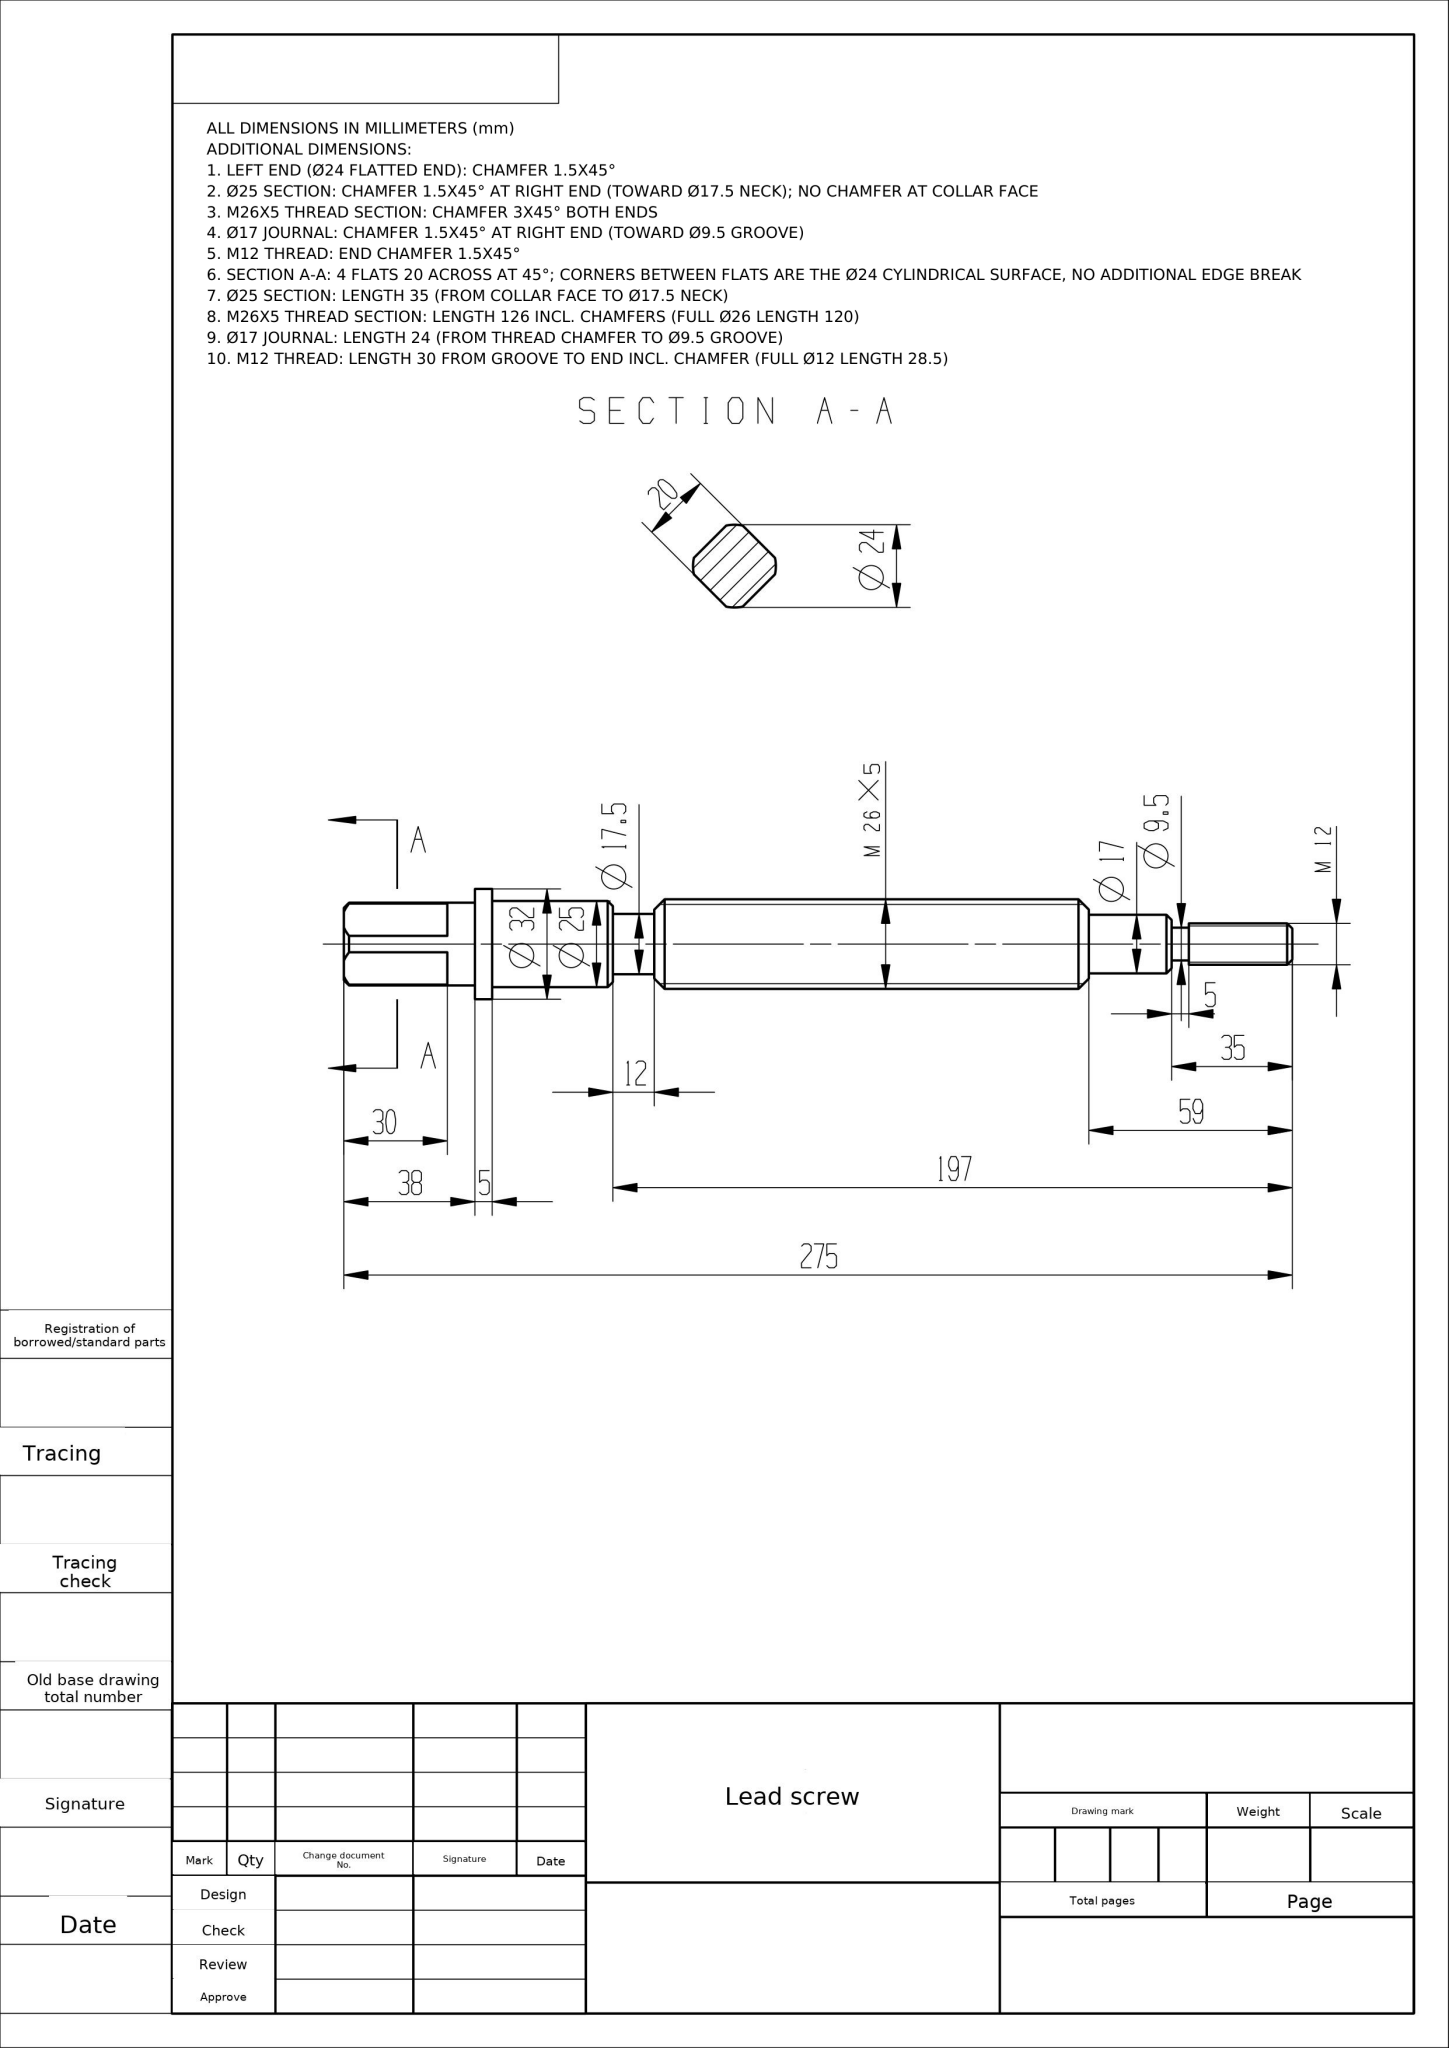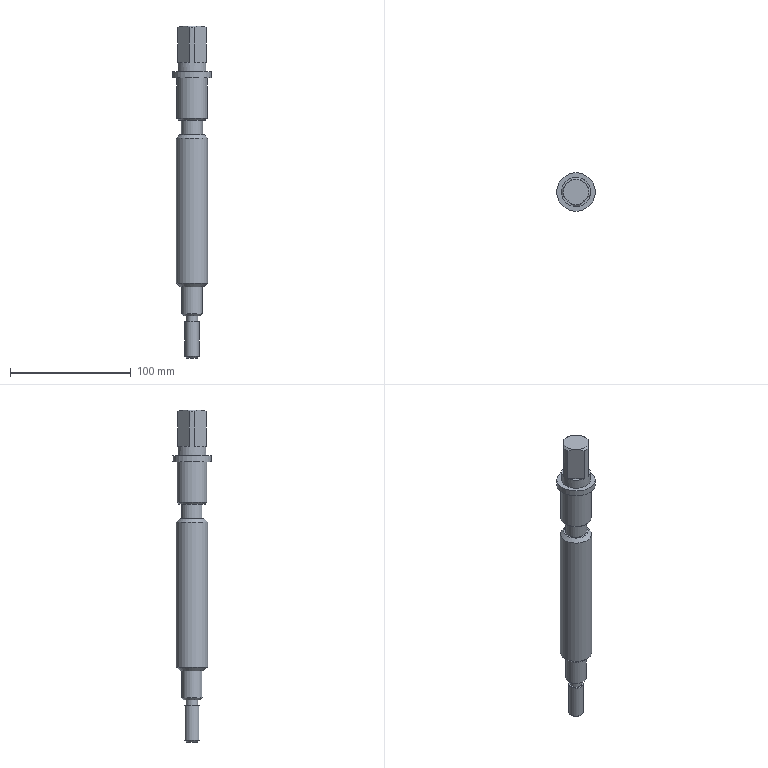Part | NX | mm | 1 solid | 34 faces | box 32 x 32 x 275 mm | volume 114323 mm3 | plane 17 | cone 9 | cylinder 8 | commonest cylinder face diameters 17.5 x1 25 x1 24 x1 32 x1 26 x1 12 x1 9.5 x1 17 x1
STEP:
#1=CARTESIAN_POINT('',(0.,0.,0.));
#2=DIRECTION('',(0.,0.,1.));
#3=DIRECTION('',(1.,0.,0.));
#4=AXIS2_PLACEMENT_3D('',#1,#2,#3);
#5=(LENGTH_UNIT()NAMED_UNIT(*)SI_UNIT(.MILLI.,.METRE.));
#6=UNCERTAINTY_MEASURE_WITH_UNIT(LENGTH_MEASURE(0.0508),#5,'','');
#7=(NAMED_UNIT(*)PLANE_ANGLE_UNIT()SI_UNIT($,.RADIAN.));
#8=PLANE_ANGLE_MEASURE_WITH_UNIT(PLANE_ANGLE_MEASURE(0.01745),#7);
#9=DIMENSIONAL_EXPONENTS(0.,0.,0.,0.,0.,0.,0.);
#10=(CONVERSION_BASED_UNIT('',#8)NAMED_UNIT(#9)PLANE_ANGLE_UNIT());
#11=(NAMED_UNIT(*)SI_UNIT($,.STERADIAN.)SOLID_ANGLE_UNIT());
#12=(GEOMETRIC_REPRESENTATION_CONTEXT(3)GLOBAL_UNCERTAINTY_ASSIGNED_CONTEXT((#6))GLOBAL_UNIT_ASSIGNED_CONTEXT((#5,#10,#11))REPRESENTATION_CONTEXT('',''));
#13=SHAPE_REPRESENTATION('',(#4),#12);
#14=CARTESIAN_POINT('',(11.,0.,155.));
#15=VERTEX_POINT('',#14);
#16=CARTESIAN_POINT('',(0.,0.,155.));
#17=DIRECTION('',(0.,0.,-1.));
#18=DIRECTION('',(1.,0.,0.));
#19=AXIS2_PLACEMENT_3D('',#16,#17,#18);
#20=CIRCLE('',#19,11.);
#21=EDGE_CURVE('',#15,#15,#20,.T.);
#22=ORIENTED_EDGE('',*,*,#21,.T.);
#23=EDGE_LOOP('',(#22));
#24=FACE_BOUND('',#23,.T.);
#25=CARTESIAN_POINT('',(8.75,0.,155.));
#26=VERTEX_POINT('',#25);
#27=CARTESIAN_POINT('',(0.,0.,155.));
#28=DIRECTION('',(0.,0.,-1.));
#29=DIRECTION('',(1.,0.,0.));
#30=AXIS2_PLACEMENT_3D('',#27,#28,#29);
#31=CIRCLE('',#30,8.75);
#32=EDGE_CURVE('',#26,#26,#31,.T.);
#33=ORIENTED_EDGE('',*,*,#32,.F.);
#34=EDGE_LOOP('',(#33));
#35=FACE_BOUND('',#34,.T.);
#36=CARTESIAN_POINT('',(0.,0.,155.));
#37=DIRECTION('',(0.,0.,1.));
#38=DIRECTION('',(1.,0.,0.));
#39=AXIS2_PLACEMENT_3D('',#36,#37,#38);
#40=PLANE('',#39);
#41=ADVANCED_FACE('',(#24,#35),#40,.F.);
#42=CARTESIAN_POINT('',(10.,0.,143.));
#43=VERTEX_POINT('',#42);
#44=CARTESIAN_POINT('',(0.,0.,143.));
#45=DIRECTION('',(0.,0.,1.));
#46=DIRECTION('',(1.,0.,0.));
#47=AXIS2_PLACEMENT_3D('',#44,#45,#46);
#48=CIRCLE('',#47,10.);
#49=EDGE_CURVE('',#43,#43,#48,.T.);
#50=ORIENTED_EDGE('',*,*,#49,.T.);
#51=EDGE_LOOP('',(#50));
#52=FACE_BOUND('',#51,.T.);
#53=CARTESIAN_POINT('',(8.75,0.,143.));
#54=VERTEX_POINT('',#53);
#55=CARTESIAN_POINT('',(0.,0.,143.));
#56=DIRECTION('',(0.,0.,-1.));
#57=DIRECTION('',(1.,0.,0.));
#58=AXIS2_PLACEMENT_3D('',#55,#56,#57);
#59=CIRCLE('',#58,8.75);
#60=EDGE_CURVE('',#54,#54,#59,.T.);
#61=ORIENTED_EDGE('',*,*,#60,.T.);
#62=EDGE_LOOP('',(#61));
#63=FACE_BOUND('',#62,.T.);
#64=CARTESIAN_POINT('',(0.,0.,143.));
#65=DIRECTION('',(0.,0.,1.));
#66=DIRECTION('',(1.,0.,0.));
#67=AXIS2_PLACEMENT_3D('',#64,#65,#66);
#68=PLANE('',#67);
#69=ADVANCED_FACE('',(#52,#63),#68,.T.);
#70=ORIENTED_EDGE('',*,*,#32,.T.);
#71=EDGE_LOOP('',(#70));
#72=FACE_BOUND('',#71,.T.);
#73=ORIENTED_EDGE('',*,*,#60,.F.);
#74=EDGE_LOOP('',(#73));
#75=FACE_BOUND('',#74,.T.);
#76=CARTESIAN_POINT('',(0.,0.,155.));
#77=DIRECTION('',(0.,0.,-1.));
#78=DIRECTION('',(-1.,0.,0.));
#79=AXIS2_PLACEMENT_3D('',#76,#77,#78);
#80=CYLINDRICAL_SURFACE('',#79,8.75);
#81=ADVANCED_FACE('',(#72,#75),#80,.T.);
#82=CARTESIAN_POINT('',(12.5,0.,156.5));
#83=VERTEX_POINT('',#82);
#84=CARTESIAN_POINT('',(0.,0.,156.5));
#85=DIRECTION('',(0.,0.,1.));
#86=DIRECTION('',(1.,0.,0.));
#87=AXIS2_PLACEMENT_3D('',#84,#85,#86);
#88=CIRCLE('',#87,12.5);
#89=EDGE_CURVE('',#83,#83,#88,.T.);
#90=ORIENTED_EDGE('',*,*,#89,.T.);
#91=EDGE_LOOP('',(#90));
#92=FACE_BOUND('',#91,.T.);
#93=CARTESIAN_POINT('',(12.5,0.,190.));
#94=VERTEX_POINT('',#93);
#95=CARTESIAN_POINT('',(0.,0.,190.));
#96=DIRECTION('',(0.,0.,-1.));
#97=DIRECTION('',(1.,0.,0.));
#98=AXIS2_PLACEMENT_3D('',#95,#96,#97);
#99=CIRCLE('',#98,12.5);
#100=EDGE_CURVE('',#94,#94,#99,.T.);
#101=ORIENTED_EDGE('',*,*,#100,.T.);
#102=EDGE_LOOP('',(#101));
#103=FACE_BOUND('',#102,.T.);
#104=CARTESIAN_POINT('',(0.,0.,155.));
#105=DIRECTION('',(0.,0.,1.));
#106=DIRECTION('',(1.,0.,0.));
#107=AXIS2_PLACEMENT_3D('',#104,#105,#106);
#108=CYLINDRICAL_SURFACE('',#107,12.5);
#109=ADVANCED_FACE('',(#92,#103),#108,.T.);
#110=CARTESIAN_POINT('',(-9.335,4.807,233.));
#111=VERTEX_POINT('',#110);
#112=CARTESIAN_POINT('',(-4.807,9.335,233.));
#113=VERTEX_POINT('',#112);
#114=CARTESIAN_POINT('',(-11.761,2.381,233.));
#115=DIRECTION('',(0.7071,0.7071,0.));
#116=VECTOR('',#115,1.);
#117=LINE('',#114,#116);
#118=EDGE_CURVE('',#111,#113,#117,.T.);
#119=ORIENTED_EDGE('',*,*,#118,.F.);
#120=CARTESIAN_POINT('',(-9.335,-4.807,233.));
#121=VERTEX_POINT('',#120);
#122=CARTESIAN_POINT('',(0.,0.,233.));
#123=DIRECTION('',(0.,0.,1.));
#124=DIRECTION('',(1.,0.,0.));
#125=AXIS2_PLACEMENT_3D('',#122,#123,#124);
#126=CIRCLE('',#125,10.5);
#127=EDGE_CURVE('',#111,#121,#126,.T.);
#128=ORIENTED_EDGE('',*,*,#127,.T.);
#129=CARTESIAN_POINT('',(-4.807,-9.335,233.));
#130=VERTEX_POINT('',#129);
#131=CARTESIAN_POINT('',(-2.381,-11.761,233.));
#132=DIRECTION('',(-0.7071,0.7071,0.));
#133=VECTOR('',#132,1.);
#134=LINE('',#131,#133);
#135=EDGE_CURVE('',#130,#121,#134,.T.);
#136=ORIENTED_EDGE('',*,*,#135,.F.);
#137=CARTESIAN_POINT('',(4.807,-9.335,233.));
#138=VERTEX_POINT('',#137);
#139=CARTESIAN_POINT('',(0.,0.,233.));
#140=DIRECTION('',(0.,0.,1.));
#141=DIRECTION('',(1.,0.,0.));
#142=AXIS2_PLACEMENT_3D('',#139,#140,#141);
#143=CIRCLE('',#142,10.5);
#144=EDGE_CURVE('',#130,#138,#143,.T.);
#145=ORIENTED_EDGE('',*,*,#144,.T.);
#146=CARTESIAN_POINT('',(9.335,-4.807,233.));
#147=VERTEX_POINT('',#146);
#148=CARTESIAN_POINT('',(11.761,-2.381,233.));
#149=DIRECTION('',(-0.7071,-0.7071,0.));
#150=VECTOR('',#149,1.);
#151=LINE('',#148,#150);
#152=EDGE_CURVE('',#147,#138,#151,.T.);
#153=ORIENTED_EDGE('',*,*,#152,.F.);
#154=CARTESIAN_POINT('',(9.335,4.807,233.));
#155=VERTEX_POINT('',#154);
#156=CARTESIAN_POINT('',(0.,0.,233.));
#157=DIRECTION('',(0.,0.,1.));
#158=DIRECTION('',(1.,0.,0.));
#159=AXIS2_PLACEMENT_3D('',#156,#157,#158);
#160=CIRCLE('',#159,10.5);
#161=EDGE_CURVE('',#147,#155,#160,.T.);
#162=ORIENTED_EDGE('',*,*,#161,.T.);
#163=CARTESIAN_POINT('',(4.807,9.335,233.));
#164=VERTEX_POINT('',#163);
#165=CARTESIAN_POINT('',(2.381,11.761,233.));
#166=DIRECTION('',(0.7071,-0.7071,0.));
#167=VECTOR('',#166,1.);
#168=LINE('',#165,#167);
#169=EDGE_CURVE('',#164,#155,#168,.T.);
#170=ORIENTED_EDGE('',*,*,#169,.F.);
#171=CARTESIAN_POINT('',(0.,0.,233.));
#172=DIRECTION('',(0.,0.,1.));
#173=DIRECTION('',(1.,0.,0.));
#174=AXIS2_PLACEMENT_3D('',#171,#172,#173);
#175=CIRCLE('',#174,10.5);
#176=EDGE_CURVE('',#164,#113,#175,.T.);
#177=ORIENTED_EDGE('',*,*,#176,.T.);
#178=EDGE_LOOP('',(#119,#128,#136,#145,#153,#162,#170,#177));
#179=FACE_OUTER_BOUND('',#178,.T.);
#180=CARTESIAN_POINT('',(0.,0.,233.));
#181=DIRECTION('',(0.,0.,1.));
#182=DIRECTION('',(1.,0.,0.));
#183=AXIS2_PLACEMENT_3D('',#180,#181,#182);
#184=PLANE('',#183);
#185=ADVANCED_FACE('',(#179),#184,.T.);
#186=CARTESIAN_POINT('',(-11.761,2.381,231.5));
#187=VERTEX_POINT('',#186);
#188=CARTESIAN_POINT('',(-11.761,2.381,231.5));
#189=CARTESIAN_POINT('',(-10.993,3.15,232.101));
#190=CARTESIAN_POINT('',(-10.184,3.958,232.634));
#191=CARTESIAN_POINT('',(-9.335,4.807,233.));
#192=B_SPLINE_CURVE_WITH_KNOTS('',3,(#188,#189,#190,#191),.UNSPECIFIED.,.F.,.F.,(4,4),(0.,1.),.UNSPECIFIED.);
#193=EDGE_CURVE('',#187,#111,#192,.T.);
#194=ORIENTED_EDGE('',*,*,#193,.F.);
#195=CARTESIAN_POINT('',(-11.761,-2.381,231.5));
#196=VERTEX_POINT('',#195);
#197=CARTESIAN_POINT('',(0.,0.,231.5));
#198=DIRECTION('',(0.,0.,-1.));
#199=DIRECTION('',(1.,0.,0.));
#200=AXIS2_PLACEMENT_3D('',#197,#198,#199);
#201=CIRCLE('',#200,12.);
#202=EDGE_CURVE('',#196,#187,#201,.T.);
#203=ORIENTED_EDGE('',*,*,#202,.F.);
#204=CARTESIAN_POINT('',(-9.335,-4.807,233.));
#205=CARTESIAN_POINT('',(-10.178,-3.964,232.636));
#206=CARTESIAN_POINT('',(-10.993,-3.149,232.101));
#207=CARTESIAN_POINT('',(-11.761,-2.381,231.5));
#208=B_SPLINE_CURVE_WITH_KNOTS('',3,(#204,#205,#206,#207),.UNSPECIFIED.,.F.,.F.,(4,4),(0.,1.),.UNSPECIFIED.);
#209=EDGE_CURVE('',#121,#196,#208,.T.);
#210=ORIENTED_EDGE('',*,*,#209,.F.);
#211=ORIENTED_EDGE('',*,*,#127,.F.);
#212=EDGE_LOOP('',(#194,#203,#210,#211));
#213=FACE_OUTER_BOUND('',#212,.T.);
#214=CARTESIAN_POINT('',(0.,0.,233.));
#215=DIRECTION('',(0.,0.,-1.));
#216=DIRECTION('',(-1.,0.,-0.));
#217=AXIS2_PLACEMENT_3D('',#214,#215,#216);
#218=CONICAL_SURFACE('',#217,10.5,45.);
#219=ADVANCED_FACE('',(#213),#218,.T.);
#220=CARTESIAN_POINT('',(-11.761,-2.381,203.));
#221=VERTEX_POINT('',#220);
#222=CARTESIAN_POINT('',(-2.381,-11.761,203.));
#223=VERTEX_POINT('',#222);
#224=CARTESIAN_POINT('',(-2.381,-11.761,203.));
#225=DIRECTION('',(0.7071,-0.7071,0.));
#226=VECTOR('',#225,1.);
#227=LINE('',#224,#226);
#228=EDGE_CURVE('',#221,#223,#227,.T.);
#229=ORIENTED_EDGE('',*,*,#228,.F.);
#230=CARTESIAN_POINT('',(0.,0.,203.));
#231=DIRECTION('',(0.,0.,1.));
#232=DIRECTION('',(-1.,-0.,0.));
#233=AXIS2_PLACEMENT_3D('',#230,#231,#232);
#234=CIRCLE('',#233,12.);
#235=EDGE_CURVE('',#221,#223,#234,.T.);
#236=ORIENTED_EDGE('',*,*,#235,.T.);
#237=EDGE_LOOP('',(#229,#236));
#238=FACE_OUTER_BOUND('',#237,.T.);
#239=CARTESIAN_POINT('',(0.,0.,203.));
#240=DIRECTION('',(0.,0.,1.));
#241=DIRECTION('',(-1.,-0.,0.));
#242=AXIS2_PLACEMENT_3D('',#239,#240,#241);
#243=PLANE('',#242);
#244=ADVANCED_FACE('',(#238),#243,.T.);
#245=CARTESIAN_POINT('',(-2.381,-11.761,231.5));
#246=VERTEX_POINT('',#245);
#247=CARTESIAN_POINT('',(-2.381,-11.761,231.5));
#248=CARTESIAN_POINT('',(-3.15,-10.993,232.101));
#249=CARTESIAN_POINT('',(-3.958,-10.184,232.634));
#250=CARTESIAN_POINT('',(-4.807,-9.335,233.));
#251=B_SPLINE_CURVE_WITH_KNOTS('',3,(#247,#248,#249,#250),.UNSPECIFIED.,.F.,.F.,(4,4),(0.,1.),.UNSPECIFIED.);
#252=EDGE_CURVE('',#246,#130,#251,.T.);
#253=ORIENTED_EDGE('',*,*,#252,.T.);
#254=ORIENTED_EDGE('',*,*,#135,.T.);
#255=ORIENTED_EDGE('',*,*,#209,.T.);
#256=CARTESIAN_POINT('',(-11.761,-2.381,203.));
#257=DIRECTION('',(0.,0.,1.));
#258=VECTOR('',#257,1.);
#259=LINE('',#256,#258);
#260=EDGE_CURVE('',#221,#196,#259,.T.);
#261=ORIENTED_EDGE('',*,*,#260,.F.);
#262=ORIENTED_EDGE('',*,*,#228,.T.);
#263=CARTESIAN_POINT('',(-2.381,-11.761,203.));
#264=DIRECTION('',(0.,0.,-1.));
#265=VECTOR('',#264,1.);
#266=LINE('',#263,#265);
#267=EDGE_CURVE('',#246,#223,#266,.T.);
#268=ORIENTED_EDGE('',*,*,#267,.F.);
#269=EDGE_LOOP('',(#253,#254,#255,#261,#262,#268));
#270=FACE_OUTER_BOUND('',#269,.T.);
#271=CARTESIAN_POINT('',(-2.381,-11.761,203.));
#272=DIRECTION('',(0.7071,0.7071,0.));
#273=DIRECTION('',(-0.7071,0.7071,0.));
#274=AXIS2_PLACEMENT_3D('',#271,#272,#273);
#275=PLANE('',#274);
#276=ADVANCED_FACE('',(#270),#275,.F.);
#277=ORIENTED_EDGE('',*,*,#252,.F.);
#278=CARTESIAN_POINT('',(2.381,-11.761,231.5));
#279=VERTEX_POINT('',#278);
#280=CARTESIAN_POINT('',(0.,0.,231.5));
#281=DIRECTION('',(0.,0.,-1.));
#282=DIRECTION('',(1.,0.,0.));
#283=AXIS2_PLACEMENT_3D('',#280,#281,#282);
#284=CIRCLE('',#283,12.);
#285=EDGE_CURVE('',#279,#246,#284,.T.);
#286=ORIENTED_EDGE('',*,*,#285,.F.);
#287=CARTESIAN_POINT('',(4.807,-9.335,233.));
#288=CARTESIAN_POINT('',(3.964,-10.178,232.636));
#289=CARTESIAN_POINT('',(3.149,-10.993,232.101));
#290=CARTESIAN_POINT('',(2.381,-11.761,231.5));
#291=B_SPLINE_CURVE_WITH_KNOTS('',3,(#287,#288,#289,#290),.UNSPECIFIED.,.F.,.F.,(4,4),(0.,1.),.UNSPECIFIED.);
#292=EDGE_CURVE('',#138,#279,#291,.T.);
#293=ORIENTED_EDGE('',*,*,#292,.F.);
#294=ORIENTED_EDGE('',*,*,#144,.F.);
#295=EDGE_LOOP('',(#277,#286,#293,#294));
#296=FACE_OUTER_BOUND('',#295,.T.);
#297=CARTESIAN_POINT('',(0.,0.,233.));
#298=DIRECTION('',(0.,0.,-1.));
#299=DIRECTION('',(-1.,0.,-0.));
#300=AXIS2_PLACEMENT_3D('',#297,#298,#299);
#301=CONICAL_SURFACE('',#300,10.5,45.);
#302=ADVANCED_FACE('',(#296),#301,.T.);
#303=CARTESIAN_POINT('',(2.381,-11.761,203.));
#304=VERTEX_POINT('',#303);
#305=CARTESIAN_POINT('',(11.761,-2.381,203.));
#306=VERTEX_POINT('',#305);
#307=CARTESIAN_POINT('',(11.761,-2.381,203.));
#308=DIRECTION('',(0.7071,0.7071,0.));
#309=VECTOR('',#308,1.);
#310=LINE('',#307,#309);
#311=EDGE_CURVE('',#304,#306,#310,.T.);
#312=ORIENTED_EDGE('',*,*,#311,.F.);
#313=CARTESIAN_POINT('',(0.,0.,203.));
#314=DIRECTION('',(0.,0.,1.));
#315=DIRECTION('',(0.,-1.,0.));
#316=AXIS2_PLACEMENT_3D('',#313,#314,#315);
#317=CIRCLE('',#316,12.);
#318=EDGE_CURVE('',#304,#306,#317,.T.);
#319=ORIENTED_EDGE('',*,*,#318,.T.);
#320=EDGE_LOOP('',(#312,#319));
#321=FACE_OUTER_BOUND('',#320,.T.);
#322=CARTESIAN_POINT('',(0.,0.,203.));
#323=DIRECTION('',(0.,0.,1.));
#324=DIRECTION('',(0.,-1.,0.));
#325=AXIS2_PLACEMENT_3D('',#322,#323,#324);
#326=PLANE('',#325);
#327=ADVANCED_FACE('',(#321),#326,.T.);
#328=CARTESIAN_POINT('',(11.761,-2.381,231.5));
#329=VERTEX_POINT('',#328);
#330=CARTESIAN_POINT('',(11.761,-2.381,231.5));
#331=CARTESIAN_POINT('',(10.993,-3.15,232.101));
#332=CARTESIAN_POINT('',(10.184,-3.958,232.634));
#333=CARTESIAN_POINT('',(9.335,-4.807,233.));
#334=B_SPLINE_CURVE_WITH_KNOTS('',3,(#330,#331,#332,#333),.UNSPECIFIED.,.F.,.F.,(4,4),(0.,1.),.UNSPECIFIED.);
#335=EDGE_CURVE('',#329,#147,#334,.T.);
#336=ORIENTED_EDGE('',*,*,#335,.T.);
#337=ORIENTED_EDGE('',*,*,#152,.T.);
#338=ORIENTED_EDGE('',*,*,#292,.T.);
#339=CARTESIAN_POINT('',(2.381,-11.761,203.));
#340=DIRECTION('',(0.,0.,1.));
#341=VECTOR('',#340,1.);
#342=LINE('',#339,#341);
#343=EDGE_CURVE('',#304,#279,#342,.T.);
#344=ORIENTED_EDGE('',*,*,#343,.F.);
#345=ORIENTED_EDGE('',*,*,#311,.T.);
#346=CARTESIAN_POINT('',(11.761,-2.381,203.));
#347=DIRECTION('',(0.,0.,-1.));
#348=VECTOR('',#347,1.);
#349=LINE('',#346,#348);
#350=EDGE_CURVE('',#329,#306,#349,.T.);
#351=ORIENTED_EDGE('',*,*,#350,.F.);
#352=EDGE_LOOP('',(#336,#337,#338,#344,#345,#351));
#353=FACE_OUTER_BOUND('',#352,.T.);
#354=CARTESIAN_POINT('',(11.761,-2.381,203.));
#355=DIRECTION('',(-0.7071,0.7071,0.));
#356=DIRECTION('',(-0.7071,-0.7071,0.));
#357=AXIS2_PLACEMENT_3D('',#354,#355,#356);
#358=PLANE('',#357);
#359=ADVANCED_FACE('',(#353),#358,.F.);
#360=ORIENTED_EDGE('',*,*,#335,.F.);
#361=CARTESIAN_POINT('',(11.761,2.381,231.5));
#362=VERTEX_POINT('',#361);
#363=CARTESIAN_POINT('',(0.,0.,231.5));
#364=DIRECTION('',(0.,0.,-1.));
#365=DIRECTION('',(1.,0.,0.));
#366=AXIS2_PLACEMENT_3D('',#363,#364,#365);
#367=CIRCLE('',#366,12.);
#368=EDGE_CURVE('',#362,#329,#367,.T.);
#369=ORIENTED_EDGE('',*,*,#368,.F.);
#370=CARTESIAN_POINT('',(9.335,4.807,233.));
#371=CARTESIAN_POINT('',(10.178,3.964,232.636));
#372=CARTESIAN_POINT('',(10.993,3.149,232.101));
#373=CARTESIAN_POINT('',(11.761,2.381,231.5));
#374=B_SPLINE_CURVE_WITH_KNOTS('',3,(#370,#371,#372,#373),.UNSPECIFIED.,.F.,.F.,(4,4),(0.,1.),.UNSPECIFIED.);
#375=EDGE_CURVE('',#155,#362,#374,.T.);
#376=ORIENTED_EDGE('',*,*,#375,.F.);
#377=ORIENTED_EDGE('',*,*,#161,.F.);
#378=EDGE_LOOP('',(#360,#369,#376,#377));
#379=FACE_OUTER_BOUND('',#378,.T.);
#380=CARTESIAN_POINT('',(0.,0.,233.));
#381=DIRECTION('',(0.,0.,-1.));
#382=DIRECTION('',(-1.,0.,-0.));
#383=AXIS2_PLACEMENT_3D('',#380,#381,#382);
#384=CONICAL_SURFACE('',#383,10.5,45.);
#385=ADVANCED_FACE('',(#379),#384,.T.);
#386=CARTESIAN_POINT('',(11.761,2.381,203.));
#387=VERTEX_POINT('',#386);
#388=CARTESIAN_POINT('',(2.381,11.761,203.));
#389=VERTEX_POINT('',#388);
#390=CARTESIAN_POINT('',(2.381,11.761,203.));
#391=DIRECTION('',(-0.7071,0.7071,0.));
#392=VECTOR('',#391,1.);
#393=LINE('',#390,#392);
#394=EDGE_CURVE('',#387,#389,#393,.T.);
#395=ORIENTED_EDGE('',*,*,#394,.F.);
#396=CARTESIAN_POINT('',(0.,0.,203.));
#397=DIRECTION('',(0.,0.,1.));
#398=DIRECTION('',(1.,0.,0.));
#399=AXIS2_PLACEMENT_3D('',#396,#397,#398);
#400=CIRCLE('',#399,12.);
#401=EDGE_CURVE('',#387,#389,#400,.T.);
#402=ORIENTED_EDGE('',*,*,#401,.T.);
#403=EDGE_LOOP('',(#395,#402));
#404=FACE_OUTER_BOUND('',#403,.T.);
#405=CARTESIAN_POINT('',(0.,0.,203.));
#406=DIRECTION('',(0.,0.,1.));
#407=DIRECTION('',(1.,0.,0.));
#408=AXIS2_PLACEMENT_3D('',#405,#406,#407);
#409=PLANE('',#408);
#410=ADVANCED_FACE('',(#404),#409,.T.);
#411=CARTESIAN_POINT('',(2.381,11.761,231.5));
#412=VERTEX_POINT('',#411);
#413=CARTESIAN_POINT('',(2.381,11.761,231.5));
#414=CARTESIAN_POINT('',(3.15,10.993,232.101));
#415=CARTESIAN_POINT('',(3.958,10.184,232.634));
#416=CARTESIAN_POINT('',(4.807,9.335,233.));
#417=B_SPLINE_CURVE_WITH_KNOTS('',3,(#413,#414,#415,#416),.UNSPECIFIED.,.F.,.F.,(4,4),(0.,1.),.UNSPECIFIED.);
#418=EDGE_CURVE('',#412,#164,#417,.T.);
#419=ORIENTED_EDGE('',*,*,#418,.T.);
#420=ORIENTED_EDGE('',*,*,#169,.T.);
#421=ORIENTED_EDGE('',*,*,#375,.T.);
#422=CARTESIAN_POINT('',(11.761,2.381,203.));
#423=DIRECTION('',(0.,0.,1.));
#424=VECTOR('',#423,1.);
#425=LINE('',#422,#424);
#426=EDGE_CURVE('',#387,#362,#425,.T.);
#427=ORIENTED_EDGE('',*,*,#426,.F.);
#428=ORIENTED_EDGE('',*,*,#394,.T.);
#429=CARTESIAN_POINT('',(2.381,11.761,203.));
#430=DIRECTION('',(0.,0.,-1.));
#431=VECTOR('',#430,1.);
#432=LINE('',#429,#431);
#433=EDGE_CURVE('',#412,#389,#432,.T.);
#434=ORIENTED_EDGE('',*,*,#433,.F.);
#435=EDGE_LOOP('',(#419,#420,#421,#427,#428,#434));
#436=FACE_OUTER_BOUND('',#435,.T.);
#437=CARTESIAN_POINT('',(2.381,11.761,203.));
#438=DIRECTION('',(-0.7071,-0.7071,0.));
#439=DIRECTION('',(0.7071,-0.7071,0.));
#440=AXIS2_PLACEMENT_3D('',#437,#438,#439);
#441=PLANE('',#440);
#442=ADVANCED_FACE('',(#436),#441,.F.);
#443=CARTESIAN_POINT('',(-2.381,11.761,231.5));
#444=VERTEX_POINT('',#443);
#445=CARTESIAN_POINT('',(-4.807,9.335,233.));
#446=CARTESIAN_POINT('',(-3.964,10.178,232.636));
#447=CARTESIAN_POINT('',(-3.149,10.993,232.101));
#448=CARTESIAN_POINT('',(-2.381,11.761,231.5));
#449=B_SPLINE_CURVE_WITH_KNOTS('',3,(#445,#446,#447,#448),.UNSPECIFIED.,.F.,.F.,(4,4),(0.,1.),.UNSPECIFIED.);
#450=EDGE_CURVE('',#113,#444,#449,.T.);
#451=ORIENTED_EDGE('',*,*,#450,.F.);
#452=ORIENTED_EDGE('',*,*,#176,.F.);
#453=ORIENTED_EDGE('',*,*,#418,.F.);
#454=CARTESIAN_POINT('',(0.,0.,231.5));
#455=DIRECTION('',(0.,0.,-1.));
#456=DIRECTION('',(1.,0.,0.));
#457=AXIS2_PLACEMENT_3D('',#454,#455,#456);
#458=CIRCLE('',#457,12.);
#459=EDGE_CURVE('',#444,#412,#458,.T.);
#460=ORIENTED_EDGE('',*,*,#459,.F.);
#461=EDGE_LOOP('',(#451,#452,#453,#460));
#462=FACE_OUTER_BOUND('',#461,.T.);
#463=CARTESIAN_POINT('',(0.,0.,233.));
#464=DIRECTION('',(0.,0.,-1.));
#465=DIRECTION('',(-1.,0.,-0.));
#466=AXIS2_PLACEMENT_3D('',#463,#464,#465);
#467=CONICAL_SURFACE('',#466,10.5,45.);
#468=ADVANCED_FACE('',(#462),#467,.T.);
#469=ORIENTED_EDGE('',*,*,#193,.T.);
#470=ORIENTED_EDGE('',*,*,#118,.T.);
#471=ORIENTED_EDGE('',*,*,#450,.T.);
#472=CARTESIAN_POINT('',(-2.381,11.761,203.));
#473=VERTEX_POINT('',#472);
#474=CARTESIAN_POINT('',(-2.381,11.761,203.));
#475=DIRECTION('',(0.,0.,1.));
#476=VECTOR('',#475,1.);
#477=LINE('',#474,#476);
#478=EDGE_CURVE('',#473,#444,#477,.T.);
#479=ORIENTED_EDGE('',*,*,#478,.F.);
#480=CARTESIAN_POINT('',(-11.761,2.381,203.));
#481=VERTEX_POINT('',#480);
#482=CARTESIAN_POINT('',(-11.761,2.381,203.));
#483=DIRECTION('',(-0.7071,-0.7071,0.));
#484=VECTOR('',#483,1.);
#485=LINE('',#482,#484);
#486=EDGE_CURVE('',#473,#481,#485,.T.);
#487=ORIENTED_EDGE('',*,*,#486,.T.);
#488=CARTESIAN_POINT('',(-11.761,2.381,203.));
#489=DIRECTION('',(0.,0.,-1.));
#490=VECTOR('',#489,1.);
#491=LINE('',#488,#490);
#492=EDGE_CURVE('',#187,#481,#491,.T.);
#493=ORIENTED_EDGE('',*,*,#492,.F.);
#494=EDGE_LOOP('',(#469,#470,#471,#479,#487,#493));
#495=FACE_OUTER_BOUND('',#494,.T.);
#496=CARTESIAN_POINT('',(-11.761,2.381,203.));
#497=DIRECTION('',(0.7071,-0.7071,0.));
#498=DIRECTION('',(0.7071,0.7071,0.));
#499=AXIS2_PLACEMENT_3D('',#496,#497,#498);
#500=PLANE('',#499);
#501=ADVANCED_FACE('',(#495),#500,.F.);
#502=ORIENTED_EDGE('',*,*,#486,.F.);
#503=CARTESIAN_POINT('',(0.,0.,203.));
#504=DIRECTION('',(0.,0.,1.));
#505=DIRECTION('',(-0.,1.,0.));
#506=AXIS2_PLACEMENT_3D('',#503,#504,#505);
#507=CIRCLE('',#506,12.);
#508=EDGE_CURVE('',#473,#481,#507,.T.);
#509=ORIENTED_EDGE('',*,*,#508,.T.);
#510=EDGE_LOOP('',(#502,#509));
#511=FACE_OUTER_BOUND('',#510,.T.);
#512=CARTESIAN_POINT('',(0.,0.,203.));
#513=DIRECTION('',(0.,0.,1.));
#514=DIRECTION('',(-0.,1.,0.));
#515=AXIS2_PLACEMENT_3D('',#512,#513,#514);
#516=PLANE('',#515);
#517=ADVANCED_FACE('',(#511),#516,.T.);
#518=ORIENTED_EDGE('',*,*,#508,.F.);
#519=ORIENTED_EDGE('',*,*,#478,.T.);
#520=ORIENTED_EDGE('',*,*,#459,.T.);
#521=ORIENTED_EDGE('',*,*,#433,.T.);
#522=ORIENTED_EDGE('',*,*,#401,.F.);
#523=ORIENTED_EDGE('',*,*,#426,.T.);
#524=ORIENTED_EDGE('',*,*,#368,.T.);
#525=ORIENTED_EDGE('',*,*,#350,.T.);
#526=ORIENTED_EDGE('',*,*,#318,.F.);
#527=ORIENTED_EDGE('',*,*,#343,.T.);
#528=ORIENTED_EDGE('',*,*,#285,.T.);
#529=ORIENTED_EDGE('',*,*,#267,.T.);
#530=ORIENTED_EDGE('',*,*,#235,.F.);
#531=ORIENTED_EDGE('',*,*,#260,.T.);
#532=ORIENTED_EDGE('',*,*,#202,.T.);
#533=ORIENTED_EDGE('',*,*,#492,.T.);
#534=EDGE_LOOP('',(#518,#519,#520,#521,#522,#523,#524,#525,#526,#527,#528,#529,#530,#531,#532,#533));
#535=FACE_BOUND('',#534,.T.);
#536=CARTESIAN_POINT('',(12.,0.,195.));
#537=VERTEX_POINT('',#536);
#538=CARTESIAN_POINT('',(0.,0.,195.));
#539=DIRECTION('',(0.,0.,1.));
#540=DIRECTION('',(1.,0.,0.));
#541=AXIS2_PLACEMENT_3D('',#538,#539,#540);
#542=CIRCLE('',#541,12.);
#543=EDGE_CURVE('',#537,#537,#542,.T.);
#544=ORIENTED_EDGE('',*,*,#543,.T.);
#545=EDGE_LOOP('',(#544));
#546=FACE_BOUND('',#545,.T.);
#547=CARTESIAN_POINT('',(0.,0.,233.));
#548=DIRECTION('',(0.,0.,-1.));
#549=DIRECTION('',(-1.,0.,0.));
#550=AXIS2_PLACEMENT_3D('',#547,#548,#549);
#551=CYLINDRICAL_SURFACE('',#550,12.);
#552=ADVANCED_FACE('',(#535,#546),#551,.T.);
#553=ORIENTED_EDGE('',*,*,#543,.F.);
#554=EDGE_LOOP('',(#553));
#555=FACE_BOUND('',#554,.T.);
#556=CARTESIAN_POINT('',(16.,0.,195.));
#557=VERTEX_POINT('',#556);
#558=CARTESIAN_POINT('',(0.,0.,195.));
#559=DIRECTION('',(0.,0.,1.));
#560=DIRECTION('',(1.,0.,0.));
#561=AXIS2_PLACEMENT_3D('',#558,#559,#560);
#562=CIRCLE('',#561,16.);
#563=EDGE_CURVE('',#557,#557,#562,.T.);
#564=ORIENTED_EDGE('',*,*,#563,.T.);
#565=EDGE_LOOP('',(#564));
#566=FACE_BOUND('',#565,.T.);
#567=CARTESIAN_POINT('',(0.,0.,195.));
#568=DIRECTION('',(0.,0.,1.));
#569=DIRECTION('',(1.,0.,0.));
#570=AXIS2_PLACEMENT_3D('',#567,#568,#569);
#571=PLANE('',#570);
#572=ADVANCED_FACE('',(#555,#566),#571,.T.);
#573=ORIENTED_EDGE('',*,*,#563,.F.);
#574=EDGE_LOOP('',(#573));
#575=FACE_BOUND('',#574,.T.);
#576=CARTESIAN_POINT('',(16.,0.,190.));
#577=VERTEX_POINT('',#576);
#578=CARTESIAN_POINT('',(0.,0.,190.));
#579=DIRECTION('',(0.,0.,1.));
#580=DIRECTION('',(1.,0.,0.));
#581=AXIS2_PLACEMENT_3D('',#578,#579,#580);
#582=CIRCLE('',#581,16.);
#583=EDGE_CURVE('',#577,#577,#582,.T.);
#584=ORIENTED_EDGE('',*,*,#583,.T.);
#585=EDGE_LOOP('',(#584));
#586=FACE_BOUND('',#585,.T.);
#587=CARTESIAN_POINT('',(0.,0.,195.));
#588=DIRECTION('',(0.,0.,-1.));
#589=DIRECTION('',(-1.,0.,0.));
#590=AXIS2_PLACEMENT_3D('',#587,#588,#589);
#591=CYLINDRICAL_SURFACE('',#590,16.);
#592=ADVANCED_FACE('',(#575,#586),#591,.T.);
#593=ORIENTED_EDGE('',*,*,#100,.F.);
#594=EDGE_LOOP('',(#593));
#595=FACE_BOUND('',#594,.T.);
#596=ORIENTED_EDGE('',*,*,#583,.F.);
#597=EDGE_LOOP('',(#596));
#598=FACE_BOUND('',#597,.T.);
#599=CARTESIAN_POINT('',(0.,0.,190.));
#600=DIRECTION('',(0.,0.,1.));
#601=DIRECTION('',(1.,0.,0.));
#602=AXIS2_PLACEMENT_3D('',#599,#600,#601);
#603=PLANE('',#602);
#604=ADVANCED_FACE('',(#595,#598),#603,.F.);
#605=ORIENTED_EDGE('',*,*,#89,.F.);
#606=EDGE_LOOP('',(#605));
#607=FACE_BOUND('',#606,.T.);
#608=ORIENTED_EDGE('',*,*,#21,.F.);
#609=EDGE_LOOP('',(#608));
#610=FACE_BOUND('',#609,.T.);
#611=CARTESIAN_POINT('',(0.,0.,155.));
#612=DIRECTION('',(0.,0.,1.));
#613=DIRECTION('',(1.,0.,0.));
#614=AXIS2_PLACEMENT_3D('',#611,#612,#613);
#615=CONICAL_SURFACE('',#614,11.,45.);
#616=ADVANCED_FACE('',(#607,#610),#615,.T.);
#617=CARTESIAN_POINT('',(13.,0.,20.));
#618=VERTEX_POINT('',#617);
#619=CARTESIAN_POINT('',(0.,0.,20.));
#620=DIRECTION('',(0.,0.,1.));
#621=DIRECTION('',(1.,0.,0.));
#622=AXIS2_PLACEMENT_3D('',#619,#620,#621);
#623=CIRCLE('',#622,13.);
#624=EDGE_CURVE('',#618,#618,#623,.T.);
#625=ORIENTED_EDGE('',*,*,#624,.T.);
#626=EDGE_LOOP('',(#625));
#627=FACE_BOUND('',#626,.T.);
#628=CARTESIAN_POINT('',(13.,0.,140.));
#629=VERTEX_POINT('',#628);
#630=CARTESIAN_POINT('',(0.,0.,140.));
#631=DIRECTION('',(0.,0.,-1.));
#632=DIRECTION('',(1.,0.,0.));
#633=AXIS2_PLACEMENT_3D('',#630,#631,#632);
#634=CIRCLE('',#633,13.);
#635=EDGE_CURVE('',#629,#629,#634,.T.);
#636=ORIENTED_EDGE('',*,*,#635,.T.);
#637=EDGE_LOOP('',(#636));
#638=FACE_BOUND('',#637,.T.);
#639=CARTESIAN_POINT('',(0.,0.,143.));
#640=DIRECTION('',(0.,0.,-1.));
#641=DIRECTION('',(-1.,0.,0.));
#642=AXIS2_PLACEMENT_3D('',#639,#640,#641);
#643=CYLINDRICAL_SURFACE('',#642,13.);
#644=ADVANCED_FACE('',(#627,#638),#643,.T.);
#645=CARTESIAN_POINT('',(-4.5,0.,-42.));
#646=VERTEX_POINT('',#645);
#647=CARTESIAN_POINT('',(0.,0.,-42.));
#648=DIRECTION('',(0.,0.,-1.));
#649=DIRECTION('',(-1.,0.,0.));
#650=AXIS2_PLACEMENT_3D('',#647,#648,#649);
#651=CIRCLE('',#650,4.5);
#652=EDGE_CURVE('',#646,#646,#651,.T.);
#653=ORIENTED_EDGE('',*,*,#652,.T.);
#654=EDGE_LOOP('',(#653));
#655=FACE_OUTER_BOUND('',#654,.T.);
#656=CARTESIAN_POINT('',(0.,0.,-42.));
#657=DIRECTION('',(0.,0.,-1.));
#658=DIRECTION('',(-1.,0.,0.));
#659=AXIS2_PLACEMENT_3D('',#656,#657,#658);
#660=PLANE('',#659);
#661=ADVANCED_FACE('',(#655),#660,.T.);
#662=CARTESIAN_POINT('',(-6.,0.,-40.5));
#663=VERTEX_POINT('',#662);
#664=CARTESIAN_POINT('',(0.,0.,-40.5));
#665=DIRECTION('',(0.,0.,1.));
#666=DIRECTION('',(-1.,0.,0.));
#667=AXIS2_PLACEMENT_3D('',#664,#665,#666);
#668=CIRCLE('',#667,6.);
#669=EDGE_CURVE('',#663,#663,#668,.T.);
#670=ORIENTED_EDGE('',*,*,#669,.F.);
#671=EDGE_LOOP('',(#670));
#672=FACE_BOUND('',#671,.T.);
#673=ORIENTED_EDGE('',*,*,#652,.F.);
#674=EDGE_LOOP('',(#673));
#675=FACE_BOUND('',#674,.T.);
#676=CARTESIAN_POINT('',(0.,0.,-42.));
#677=DIRECTION('',(0.,0.,1.));
#678=DIRECTION('',(1.,0.,-0.));
#679=AXIS2_PLACEMENT_3D('',#676,#677,#678);
#680=CONICAL_SURFACE('',#679,4.5,45.);
#681=ADVANCED_FACE('',(#672,#675),#680,.T.);
#682=ORIENTED_EDGE('',*,*,#669,.T.);
#683=EDGE_LOOP('',(#682));
#684=FACE_BOUND('',#683,.T.);
#685=CARTESIAN_POINT('',(-6.,0.,-12.));
#686=VERTEX_POINT('',#685);
#687=CARTESIAN_POINT('',(0.,0.,-12.));
#688=DIRECTION('',(0.,0.,-1.));
#689=DIRECTION('',(-1.,0.,0.));
#690=AXIS2_PLACEMENT_3D('',#687,#688,#689);
#691=CIRCLE('',#690,6.);
#692=EDGE_CURVE('',#686,#686,#691,.T.);
#693=ORIENTED_EDGE('',*,*,#692,.T.);
#694=EDGE_LOOP('',(#693));
#695=FACE_BOUND('',#694,.T.);
#696=CARTESIAN_POINT('',(0.,0.,-42.));
#697=DIRECTION('',(0.,0.,1.));
#698=DIRECTION('',(1.,0.,0.));
#699=AXIS2_PLACEMENT_3D('',#696,#697,#698);
#700=CYLINDRICAL_SURFACE('',#699,6.);
#701=ADVANCED_FACE('',(#684,#695),#700,.T.);
#702=CARTESIAN_POINT('',(4.75,0.,-12.));
#703=VERTEX_POINT('',#702);
#704=CARTESIAN_POINT('',(0.,0.,-12.));
#705=DIRECTION('',(0.,0.,1.));
#706=DIRECTION('',(1.,0.,0.));
#707=AXIS2_PLACEMENT_3D('',#704,#705,#706);
#708=CIRCLE('',#707,4.75);
#709=EDGE_CURVE('',#703,#703,#708,.T.);
#710=ORIENTED_EDGE('',*,*,#709,.F.);
#711=EDGE_LOOP('',(#710));
#712=FACE_BOUND('',#711,.T.);
#713=ORIENTED_EDGE('',*,*,#692,.F.);
#714=EDGE_LOOP('',(#713));
#715=FACE_BOUND('',#714,.T.);
#716=CARTESIAN_POINT('',(0.,0.,-12.));
#717=DIRECTION('',(0.,0.,-1.));
#718=DIRECTION('',(-1.,0.,0.));
#719=AXIS2_PLACEMENT_3D('',#716,#717,#718);
#720=PLANE('',#719);
#721=ADVANCED_FACE('',(#712,#715),#720,.F.);
#722=ORIENTED_EDGE('',*,*,#709,.T.);
#723=EDGE_LOOP('',(#722));
#724=FACE_BOUND('',#723,.T.);
#725=CARTESIAN_POINT('',(4.75,0.,-7.));
#726=VERTEX_POINT('',#725);
#727=CARTESIAN_POINT('',(0.,0.,-7.));
#728=DIRECTION('',(0.,0.,-1.));
#729=DIRECTION('',(1.,0.,0.));
#730=AXIS2_PLACEMENT_3D('',#727,#728,#729);
#731=CIRCLE('',#730,4.75);
#732=EDGE_CURVE('',#726,#726,#731,.T.);
#733=ORIENTED_EDGE('',*,*,#732,.T.);
#734=EDGE_LOOP('',(#733));
#735=FACE_BOUND('',#734,.T.);
#736=CARTESIAN_POINT('',(0.,0.,-12.));
#737=DIRECTION('',(0.,0.,1.));
#738=DIRECTION('',(1.,0.,0.));
#739=AXIS2_PLACEMENT_3D('',#736,#737,#738);
#740=CYLINDRICAL_SURFACE('',#739,4.75);
#741=ADVANCED_FACE('',(#724,#735),#740,.T.);
#742=CARTESIAN_POINT('',(-7.,0.,-7.));
#743=VERTEX_POINT('',#742);
#744=CARTESIAN_POINT('',(0.,0.,-7.));
#745=DIRECTION('',(0.,0.,-1.));
#746=DIRECTION('',(-1.,0.,0.));
#747=AXIS2_PLACEMENT_3D('',#744,#745,#746);
#748=CIRCLE('',#747,7.);
#749=EDGE_CURVE('',#743,#743,#748,.T.);
#750=ORIENTED_EDGE('',*,*,#749,.T.);
#751=EDGE_LOOP('',(#750));
#752=FACE_BOUND('',#751,.T.);
#753=ORIENTED_EDGE('',*,*,#732,.F.);
#754=EDGE_LOOP('',(#753));
#755=FACE_BOUND('',#754,.T.);
#756=CARTESIAN_POINT('',(0.,0.,-7.));
#757=DIRECTION('',(0.,0.,-1.));
#758=DIRECTION('',(-1.,0.,0.));
#759=AXIS2_PLACEMENT_3D('',#756,#757,#758);
#760=PLANE('',#759);
#761=ADVANCED_FACE('',(#752,#755),#760,.T.);
#762=CARTESIAN_POINT('',(-8.5,0.,-5.5));
#763=VERTEX_POINT('',#762);
#764=CARTESIAN_POINT('',(0.,0.,-5.5));
#765=DIRECTION('',(0.,0.,1.));
#766=DIRECTION('',(-1.,0.,0.));
#767=AXIS2_PLACEMENT_3D('',#764,#765,#766);
#768=CIRCLE('',#767,8.5);
#769=EDGE_CURVE('',#763,#763,#768,.T.);
#770=ORIENTED_EDGE('',*,*,#769,.F.);
#771=EDGE_LOOP('',(#770));
#772=FACE_BOUND('',#771,.T.);
#773=ORIENTED_EDGE('',*,*,#749,.F.);
#774=EDGE_LOOP('',(#773));
#775=FACE_BOUND('',#774,.T.);
#776=CARTESIAN_POINT('',(0.,0.,-7.));
#777=DIRECTION('',(0.,0.,1.));
#778=DIRECTION('',(1.,0.,-0.));
#779=AXIS2_PLACEMENT_3D('',#776,#777,#778);
#780=CONICAL_SURFACE('',#779,7.,45.);
#781=ADVANCED_FACE('',(#772,#775),#780,.T.);
#782=ORIENTED_EDGE('',*,*,#769,.T.);
#783=EDGE_LOOP('',(#782));
#784=FACE_BOUND('',#783,.T.);
#785=CARTESIAN_POINT('',(8.5,0.,17.));
#786=VERTEX_POINT('',#785);
#787=CARTESIAN_POINT('',(0.,0.,17.));
#788=DIRECTION('',(0.,0.,-1.));
#789=DIRECTION('',(1.,0.,0.));
#790=AXIS2_PLACEMENT_3D('',#787,#788,#789);
#791=CIRCLE('',#790,8.5);
#792=EDGE_CURVE('',#786,#786,#791,.T.);
#793=ORIENTED_EDGE('',*,*,#792,.T.);
#794=EDGE_LOOP('',(#793));
#795=FACE_BOUND('',#794,.T.);
#796=CARTESIAN_POINT('',(0.,0.,-7.));
#797=DIRECTION('',(0.,0.,1.));
#798=DIRECTION('',(1.,0.,0.));
#799=AXIS2_PLACEMENT_3D('',#796,#797,#798);
#800=CYLINDRICAL_SURFACE('',#799,8.5);
#801=ADVANCED_FACE('',(#784,#795),#800,.T.);
#802=CARTESIAN_POINT('',(10.,0.,17.));
#803=VERTEX_POINT('',#802);
#804=CARTESIAN_POINT('',(0.,0.,17.));
#805=DIRECTION('',(0.,0.,-1.));
#806=DIRECTION('',(1.,0.,0.));
#807=AXIS2_PLACEMENT_3D('',#804,#805,#806);
#808=CIRCLE('',#807,10.);
#809=EDGE_CURVE('',#803,#803,#808,.T.);
#810=ORIENTED_EDGE('',*,*,#809,.T.);
#811=EDGE_LOOP('',(#810));
#812=FACE_BOUND('',#811,.T.);
#813=ORIENTED_EDGE('',*,*,#792,.F.);
#814=EDGE_LOOP('',(#813));
#815=FACE_BOUND('',#814,.T.);
#816=CARTESIAN_POINT('',(0.,0.,17.));
#817=DIRECTION('',(0.,0.,1.));
#818=DIRECTION('',(1.,0.,0.));
#819=AXIS2_PLACEMENT_3D('',#816,#817,#818);
#820=PLANE('',#819);
#821=ADVANCED_FACE('',(#812,#815),#820,.F.);
#822=ORIENTED_EDGE('',*,*,#49,.F.);
#823=EDGE_LOOP('',(#822));
#824=FACE_BOUND('',#823,.T.);
#825=ORIENTED_EDGE('',*,*,#635,.F.);
#826=EDGE_LOOP('',(#825));
#827=FACE_BOUND('',#826,.T.);
#828=CARTESIAN_POINT('',(0.,0.,140.));
#829=DIRECTION('',(0.,0.,-1.));
#830=DIRECTION('',(-1.,0.,0.));
#831=AXIS2_PLACEMENT_3D('',#828,#829,#830);
#832=CONICAL_SURFACE('',#831,13.,45.);
#833=ADVANCED_FACE('',(#824,#827),#832,.T.);
#834=ORIENTED_EDGE('',*,*,#624,.F.);
#835=EDGE_LOOP('',(#834));
#836=FACE_BOUND('',#835,.T.);
#837=ORIENTED_EDGE('',*,*,#809,.F.);
#838=EDGE_LOOP('',(#837));
#839=FACE_BOUND('',#838,.T.);
#840=CARTESIAN_POINT('',(0.,0.,17.));
#841=DIRECTION('',(0.,0.,1.));
#842=DIRECTION('',(1.,0.,-0.));
#843=AXIS2_PLACEMENT_3D('',#840,#841,#842);
#844=CONICAL_SURFACE('',#843,10.,45.);
#845=ADVANCED_FACE('',(#836,#839),#844,.T.);
#846=CLOSED_SHELL('',(#41,#69,#81,#109,#185,#219,#244,#276,#302,#327,#359,#385,#410,#442,#468,#501,#517,#552,#572,#592,#604,#616,#644,#661,#681,#701,#721,#741,#761,#781,#801,#821,#833,#845));
#847=MANIFOLD_SOLID_BREP('',#846);
#848=ADVANCED_BREP_SHAPE_REPRESENTATION('',(#847),#12);
#849=SHAPE_REPRESENTATION_RELATIONSHIP('','',#13,#848);
#850=PRESENTATION_LAYER_ASSIGNMENT('','',(#847));
#851=COLOUR_RGB('',1.,0.6,0.);
#852=FILL_AREA_STYLE_COLOUR('',#851);
#853=FILL_AREA_STYLE('',(#852));
#854=SURFACE_STYLE_FILL_AREA(#853);
#855=SURFACE_SIDE_STYLE('',(#854));
#856=SURFACE_STYLE_USAGE(.BOTH.,#855);
#857=PRESENTATION_STYLE_ASSIGNMENT((#856));
#858=STYLED_ITEM('',(#857),#847);
#859=MECHANICAL_DESIGN_GEOMETRIC_PRESENTATION_REPRESENTATION('',(#858),#12);